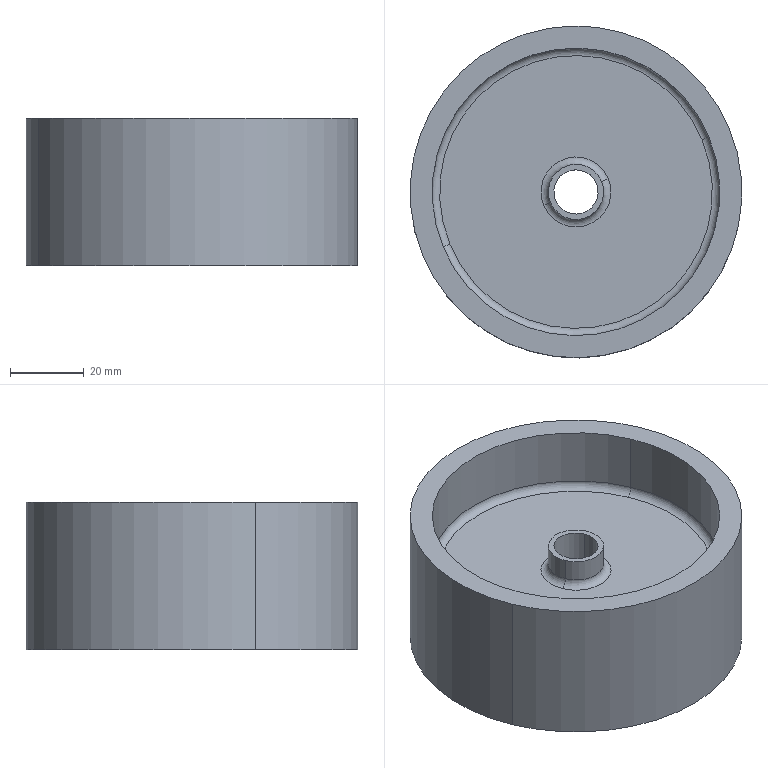Component | SolidWorks | SpringCover-2 | 1 solid | 36 faces | box 90 x 90 x 40 mm | volume 79848 mm3 | cylinder 16 | torus 12 | plane 8 | commonest cylinder face diameters 78 x4 15 x2 86 x2 18 x2 24 x2 12 x2 90 x2
build123d program:
from build123d import *

# Parameters (mm, degrees)
SKETCH1_R           = 45
SKETCH1_R_2         = 39
BOSS_EXTRUDE1_DEPTH = 20
SKETCH2_R           = 40
SKETCH2_R_2         = 6
BOSS_EXTRUDE2_DEPTH = 2
SKETCH3_R           = 12
SKETCH3_R_2         = 9
BOSS_EXTRUDE3_DEPTH = 16
BOSS_EXTRUDE4_START = 8
SKETCH5_R           = 7.5
SKETCH5_R_2         = 6
BOSS_EXTRUDE4_DEPTH = 8
FILLET1_R           = 2


with BuildPart() as part:
    # Sketch1 → Boss-Extrude1 (new, symmetric)
    with BuildSketch(Plane.XY):
        Circle(SKETCH1_R)
        Circle(SKETCH1_R_2, mode=Mode.SUBTRACT)
    extrude(amount=BOSS_EXTRUDE1_DEPTH, both=True)

    # Sketch2 → Boss-Extrude2 (add, symmetric)
    with BuildSketch(Plane.XY):
        Circle(SKETCH2_R)
        Circle(SKETCH2_R_2, mode=Mode.SUBTRACT)
    extrude(amount=BOSS_EXTRUDE2_DEPTH, both=True)

    # Sketch3 → Boss-Extrude3 (add)
    with BuildSketch(Plane.XY.offset(2)):
        Circle(SKETCH3_R)
        Circle(SKETCH3_R_2, mode=Mode.SUBTRACT)
    extrude(amount=BOSS_EXTRUDE3_DEPTH)

    # Sketch4 → Cut-Revolve1 (revolve, cut)
    with BuildSketch(Plane(origin=(0, 0, 0), x_dir=(1, 0, 0), z_dir=(0, 1, 0))):
        Polygon((-43, -14), (-33.035, -14), (-33.287, -20), (-43, -20), align=None)
    revolve(axis=Axis((0, 0, -26.979), (0, 0, 1)), mode=Mode.SUBTRACT)

    # Sketch5 → Boss-Extrude4 (add)
    with BuildSketch(Plane(origin=(0, 0, -2), x_dir=(-1, 0, 0), z_dir=(0, 0, -1)).offset(BOSS_EXTRUDE4_START)):
        with Locations(Location((0, 0, 0), (0, 0, 180))):
            Circle(SKETCH5_R)
        Circle(SKETCH5_R_2, mode=Mode.SUBTRACT)
    extrude(amount=-BOSS_EXTRUDE4_DEPTH)

    # Fillet1
    fillet1_edges = [part.edges().sort_by_distance(p)[0] for p in [
        (-39, 0, 2),
        (-39, 0, -2),
        (-9, 0, 2),
        (-12, 0, 2),
        (-39, 0, 14),
        (-7.5, 0, -2),
    ]]
    fillet(fillet1_edges, radius=FILLET1_R)


solid = part.part

# Placed as in the assembly
solid = solid.moved(Location((-15.928, -1.7, 188), (180, 0, 0)))
STEP:
#1=COLOUR_RGB('',0.7922,0.8196,0.9333);
#2=FILL_AREA_STYLE_COLOUR('',#1);
#3=FILL_AREA_STYLE('',(#2));
#4=SURFACE_STYLE_FILL_AREA(#3);
#5=SURFACE_SIDE_STYLE('',(#4));
#6=SURFACE_STYLE_USAGE(.BOTH.,#5);
#7=PRESENTATION_STYLE_ASSIGNMENT((#6));
#8=CARTESIAN_POINT('',(-1.973,-0.6249,7.323));
#9=VERTEX_POINT('',#8);
#10=CARTESIAN_POINT('',(0.7185,0.491,7.323));
#11=VERTEX_POINT('',#10);
#12=CARTESIAN_POINT('',(-0.6271,-0.06694,7.323));
#13=DIRECTION('',(0.,0.,-1.));
#14=DIRECTION('',(0.9237,0.383,0.));
#15=AXIS2_PLACEMENT_3D('',#12,#13,#14);
#16=CIRCLE('',#15,1.457);
#17=EDGE_CURVE('',#9,#11,#16,.T.);
#18=ORIENTED_EDGE('',*,*,#17,.F.);
#19=CARTESIAN_POINT('',(-2.045,-0.6551,7.244));
#20=VERTEX_POINT('',#19);
#21=CARTESIAN_POINT('',(-1.973,-0.6249,7.244));
#22=DIRECTION('',(0.383,-0.9237,0.));
#23=DIRECTION('',(0.9237,0.383,0.));
#24=AXIS2_PLACEMENT_3D('',#21,#22,#23);
#25=CIRCLE('',#24,0.07874);
#26=EDGE_CURVE('',#9,#20,#25,.T.);
#27=ORIENTED_EDGE('',*,*,#26,.T.);
#28=CARTESIAN_POINT('',(0.7912,0.5212,7.244));
#29=VERTEX_POINT('',#28);
#30=CARTESIAN_POINT('',(-0.6271,-0.06694,7.244));
#31=DIRECTION('',(0.,0.,1.));
#32=DIRECTION('',(0.9237,0.383,0.));
#33=AXIS2_PLACEMENT_3D('',#30,#31,#32);
#34=CIRCLE('',#33,1.535);
#35=EDGE_CURVE('',#29,#20,#34,.T.);
#36=ORIENTED_EDGE('',*,*,#35,.F.);
#37=CARTESIAN_POINT('',(0.7185,0.491,7.244));
#38=DIRECTION('',(-0.383,0.9237,0.));
#39=DIRECTION('',(-0.9237,-0.383,0.));
#40=AXIS2_PLACEMENT_3D('',#37,#38,#39);
#41=CIRCLE('',#40,0.07874);
#42=EDGE_CURVE('',#11,#29,#41,.T.);
#43=ORIENTED_EDGE('',*,*,#42,.F.);
#44=EDGE_LOOP('',(#18,#27,#36,#43));
#45=FACE_OUTER_BOUND('',#44,.T.);
#46=CARTESIAN_POINT('',(-0.6271,-0.06694,7.244));
#47=DIRECTION('',(0.,0.,-1.));
#48=DIRECTION('',(0.9237,0.383,0.));
#49=AXIS2_PLACEMENT_3D('',#46,#47,#48);
#50=TOROIDAL_SURFACE('',#49,1.457,0.07874);
#51=ADVANCED_FACE('',(#45),#50,.F.);
#52=CARTESIAN_POINT('',(0.7912,0.5212,6.929));
#53=VERTEX_POINT('',#52);
#54=CARTESIAN_POINT('',(-2.045,-0.6551,6.929));
#55=VERTEX_POINT('',#54);
#56=CARTESIAN_POINT('',(-0.6271,-0.06694,6.929));
#57=DIRECTION('',(0.,0.,-1.));
#58=DIRECTION('',(-0.9237,-0.383,0.));
#59=AXIS2_PLACEMENT_3D('',#56,#57,#58);
#60=CIRCLE('',#59,1.535);
#61=EDGE_CURVE('',#53,#55,#60,.T.);
#62=ORIENTED_EDGE('',*,*,#61,.F.);
#63=CARTESIAN_POINT('',(0.864,0.5514,6.85));
#64=VERTEX_POINT('',#63);
#65=CARTESIAN_POINT('',(0.864,0.5514,6.929));
#66=DIRECTION('',(0.383,-0.9237,0.));
#67=DIRECTION('',(0.9237,0.383,0.));
#68=AXIS2_PLACEMENT_3D('',#65,#66,#67);
#69=CIRCLE('',#68,0.07874);
#70=EDGE_CURVE('',#53,#64,#69,.T.);
#71=ORIENTED_EDGE('',*,*,#70,.T.);
#72=CARTESIAN_POINT('',(-2.118,-0.6852,6.85));
#73=VERTEX_POINT('',#72);
#74=CARTESIAN_POINT('',(-0.6271,-0.06694,6.85));
#75=DIRECTION('',(0.,0.,1.));
#76=DIRECTION('',(-0.9237,-0.383,0.));
#77=AXIS2_PLACEMENT_3D('',#74,#75,#76);
#78=CIRCLE('',#77,1.614);
#79=EDGE_CURVE('',#73,#64,#78,.T.);
#80=ORIENTED_EDGE('',*,*,#79,.F.);
#81=CARTESIAN_POINT('',(-2.118,-0.6852,6.929));
#82=DIRECTION('',(-0.383,0.9237,0.));
#83=DIRECTION('',(-0.9237,-0.383,0.));
#84=AXIS2_PLACEMENT_3D('',#81,#82,#83);
#85=CIRCLE('',#84,0.07874);
#86=EDGE_CURVE('',#55,#73,#85,.T.);
#87=ORIENTED_EDGE('',*,*,#86,.F.);
#88=EDGE_LOOP('',(#62,#71,#80,#87));
#89=FACE_OUTER_BOUND('',#88,.T.);
#90=CARTESIAN_POINT('',(-0.6271,-0.06694,6.929));
#91=DIRECTION('',(0.,0.,1.));
#92=DIRECTION('',(-0.9237,-0.383,0.));
#93=AXIS2_PLACEMENT_3D('',#90,#91,#92);
#94=TOROIDAL_SURFACE('',#93,1.614,0.07874);
#95=ADVANCED_FACE('',(#89),#94,.T.);
#96=CARTESIAN_POINT('',(-0.8817,-0.1725,7.323));
#97=VERTEX_POINT('',#96);
#98=CARTESIAN_POINT('',(-0.3725,0.03863,7.323));
#99=VERTEX_POINT('',#98);
#100=CARTESIAN_POINT('',(-0.6271,-0.06694,7.323));
#101=DIRECTION('',(0.,0.,-1.));
#102=DIRECTION('',(0.9237,0.383,0.));
#103=AXIS2_PLACEMENT_3D('',#100,#101,#102);
#104=CIRCLE('',#103,0.2756);
#105=EDGE_CURVE('',#97,#99,#104,.T.);
#106=ORIENTED_EDGE('',*,*,#105,.F.);
#107=CARTESIAN_POINT('',(-0.9544,-0.2027,7.244));
#108=VERTEX_POINT('',#107);
#109=CARTESIAN_POINT('',(-0.8817,-0.1725,7.244));
#110=DIRECTION('',(0.383,-0.9237,0.));
#111=DIRECTION('',(0.9237,0.383,0.));
#112=AXIS2_PLACEMENT_3D('',#109,#110,#111);
#113=CIRCLE('',#112,0.07874);
#114=EDGE_CURVE('',#97,#108,#113,.T.);
#115=ORIENTED_EDGE('',*,*,#114,.T.);
#116=CARTESIAN_POINT('',(-0.2998,0.06879,7.244));
#117=VERTEX_POINT('',#116);
#118=CARTESIAN_POINT('',(-0.6271,-0.06694,7.244));
#119=DIRECTION('',(0.,0.,1.));
#120=DIRECTION('',(0.9237,0.383,0.));
#121=AXIS2_PLACEMENT_3D('',#118,#119,#120);
#122=CIRCLE('',#121,0.3543);
#123=EDGE_CURVE('',#117,#108,#122,.T.);
#124=ORIENTED_EDGE('',*,*,#123,.F.);
#125=CARTESIAN_POINT('',(-0.3725,0.03863,7.244));
#126=DIRECTION('',(-0.383,0.9237,0.));
#127=DIRECTION('',(-0.9237,-0.383,0.));
#128=AXIS2_PLACEMENT_3D('',#125,#126,#127);
#129=CIRCLE('',#128,0.07874);
#130=EDGE_CURVE('',#99,#117,#129,.T.);
#131=ORIENTED_EDGE('',*,*,#130,.F.);
#132=EDGE_LOOP('',(#106,#115,#124,#131));
#133=FACE_OUTER_BOUND('',#132,.T.);
#134=CARTESIAN_POINT('',(-0.6271,-0.06694,7.244));
#135=DIRECTION('',(0.,0.,-1.));
#136=DIRECTION('',(0.9237,0.383,0.));
#137=AXIS2_PLACEMENT_3D('',#134,#135,#136);
#138=TOROIDAL_SURFACE('',#137,0.2756,0.07874);
#139=ADVANCED_FACE('',(#133),#138,.F.);
#140=CARTESIAN_POINT('',(-1.063,-0.2479,7.244));
#141=VERTEX_POINT('',#140);
#142=CARTESIAN_POINT('',(-0.1907,0.114,7.244));
#143=VERTEX_POINT('',#142);
#144=CARTESIAN_POINT('',(-0.6271,-0.06694,7.244));
#145=DIRECTION('',(0.,0.,-1.));
#146=DIRECTION('',(0.9237,0.383,0.));
#147=AXIS2_PLACEMENT_3D('',#144,#145,#146);
#148=CIRCLE('',#147,0.4724);
#149=EDGE_CURVE('',#141,#143,#148,.T.);
#150=ORIENTED_EDGE('',*,*,#149,.F.);
#151=CARTESIAN_POINT('',(-1.136,-0.2781,7.323));
#152=VERTEX_POINT('',#151);
#153=CARTESIAN_POINT('',(-1.136,-0.2781,7.244));
#154=DIRECTION('',(0.383,-0.9237,0.));
#155=DIRECTION('',(0.9237,0.383,0.));
#156=AXIS2_PLACEMENT_3D('',#153,#154,#155);
#157=CIRCLE('',#156,0.07874);
#158=EDGE_CURVE('',#141,#152,#157,.T.);
#159=ORIENTED_EDGE('',*,*,#158,.T.);
#160=CARTESIAN_POINT('',(-0.1179,0.1442,7.323));
#161=VERTEX_POINT('',#160);
#162=CARTESIAN_POINT('',(-0.6271,-0.06694,7.323));
#163=DIRECTION('',(0.,0.,1.));
#164=DIRECTION('',(0.9237,0.383,0.));
#165=AXIS2_PLACEMENT_3D('',#162,#163,#164);
#166=CIRCLE('',#165,0.5512);
#167=EDGE_CURVE('',#161,#152,#166,.T.);
#168=ORIENTED_EDGE('',*,*,#167,.F.);
#169=CARTESIAN_POINT('',(-0.1179,0.1442,7.244));
#170=DIRECTION('',(-0.383,0.9237,0.));
#171=DIRECTION('',(-0.9237,-0.383,0.));
#172=AXIS2_PLACEMENT_3D('',#169,#170,#171);
#173=CIRCLE('',#172,0.07874);
#174=EDGE_CURVE('',#143,#161,#173,.T.);
#175=ORIENTED_EDGE('',*,*,#174,.F.);
#176=EDGE_LOOP('',(#150,#159,#168,#175));
#177=FACE_OUTER_BOUND('',#176,.T.);
#178=CARTESIAN_POINT('',(-0.6271,-0.06694,7.244));
#179=DIRECTION('',(0.,0.,-1.));
#180=DIRECTION('',(0.9237,0.383,0.));
#181=AXIS2_PLACEMENT_3D('',#178,#179,#180);
#182=TOROIDAL_SURFACE('',#181,0.5512,0.07874);
#183=ADVANCED_FACE('',(#177),#182,.F.);
#184=CARTESIAN_POINT('',(-2.045,-0.6551,7.559));
#185=VERTEX_POINT('',#184);
#186=CARTESIAN_POINT('',(0.7912,0.5212,7.559));
#187=VERTEX_POINT('',#186);
#188=CARTESIAN_POINT('',(-0.6271,-0.06694,7.559));
#189=DIRECTION('',(0.,0.,-1.));
#190=DIRECTION('',(0.9237,0.383,0.));
#191=AXIS2_PLACEMENT_3D('',#188,#189,#190);
#192=CIRCLE('',#191,1.535);
#193=EDGE_CURVE('',#185,#187,#192,.T.);
#194=ORIENTED_EDGE('',*,*,#193,.F.);
#195=CARTESIAN_POINT('',(-1.973,-0.6249,7.48));
#196=VERTEX_POINT('',#195);
#197=CARTESIAN_POINT('',(-1.973,-0.6249,7.559));
#198=DIRECTION('',(0.383,-0.9237,0.));
#199=DIRECTION('',(0.9237,0.383,0.));
#200=AXIS2_PLACEMENT_3D('',#197,#198,#199);
#201=CIRCLE('',#200,0.07874);
#202=EDGE_CURVE('',#185,#196,#201,.T.);
#203=ORIENTED_EDGE('',*,*,#202,.T.);
#204=CARTESIAN_POINT('',(0.7185,0.491,7.48));
#205=VERTEX_POINT('',#204);
#206=CARTESIAN_POINT('',(-0.6271,-0.06694,7.48));
#207=DIRECTION('',(0.,0.,1.));
#208=DIRECTION('',(0.9237,0.383,0.));
#209=AXIS2_PLACEMENT_3D('',#206,#207,#208);
#210=CIRCLE('',#209,1.457);
#211=EDGE_CURVE('',#205,#196,#210,.T.);
#212=ORIENTED_EDGE('',*,*,#211,.F.);
#213=CARTESIAN_POINT('',(0.7185,0.491,7.559));
#214=DIRECTION('',(-0.383,0.9237,0.));
#215=DIRECTION('',(-0.9237,-0.383,0.));
#216=AXIS2_PLACEMENT_3D('',#213,#214,#215);
#217=CIRCLE('',#216,0.07874);
#218=EDGE_CURVE('',#187,#205,#217,.T.);
#219=ORIENTED_EDGE('',*,*,#218,.F.);
#220=EDGE_LOOP('',(#194,#203,#212,#219));
#221=FACE_OUTER_BOUND('',#220,.T.);
#222=CARTESIAN_POINT('',(-0.6271,-0.06694,7.559));
#223=DIRECTION('',(0.,0.,-1.));
#224=DIRECTION('',(0.9237,0.383,0.));
#225=AXIS2_PLACEMENT_3D('',#222,#223,#224);
#226=TOROIDAL_SURFACE('',#225,1.457,0.07874);
#227=ADVANCED_FACE('',(#221),#226,.F.);
#228=CARTESIAN_POINT('',(-0.9726,-0.2102,7.48));
#229=VERTEX_POINT('',#228);
#230=CARTESIAN_POINT('',(-0.2816,0.07633,7.48));
#231=VERTEX_POINT('',#230);
#232=CARTESIAN_POINT('',(-0.6271,-0.06694,7.48));
#233=DIRECTION('',(0.,0.,-1.));
#234=DIRECTION('',(0.9237,0.383,0.));
#235=AXIS2_PLACEMENT_3D('',#232,#233,#234);
#236=CIRCLE('',#235,0.374);
#237=EDGE_CURVE('',#229,#231,#236,.T.);
#238=ORIENTED_EDGE('',*,*,#237,.F.);
#239=CARTESIAN_POINT('',(-0.8998,-0.18,7.559));
#240=VERTEX_POINT('',#239);
#241=CARTESIAN_POINT('',(-0.9726,-0.2102,7.559));
#242=DIRECTION('',(0.383,-0.9237,0.));
#243=DIRECTION('',(0.9237,0.383,0.));
#244=AXIS2_PLACEMENT_3D('',#241,#242,#243);
#245=CIRCLE('',#244,0.07874);
#246=EDGE_CURVE('',#229,#240,#245,.T.);
#247=ORIENTED_EDGE('',*,*,#246,.T.);
#248=CARTESIAN_POINT('',(-0.3543,0.04617,7.559));
#249=VERTEX_POINT('',#248);
#250=CARTESIAN_POINT('',(-0.6271,-0.06694,7.559));
#251=DIRECTION('',(0.,0.,1.));
#252=DIRECTION('',(0.9237,0.383,0.));
#253=AXIS2_PLACEMENT_3D('',#250,#251,#252);
#254=CIRCLE('',#253,0.2953);
#255=EDGE_CURVE('',#249,#240,#254,.T.);
#256=ORIENTED_EDGE('',*,*,#255,.F.);
#257=CARTESIAN_POINT('',(-0.2816,0.07633,7.559));
#258=DIRECTION('',(-0.383,0.9237,0.));
#259=DIRECTION('',(-0.9237,-0.383,0.));
#260=AXIS2_PLACEMENT_3D('',#257,#258,#259);
#261=CIRCLE('',#260,0.07874);
#262=EDGE_CURVE('',#231,#249,#261,.T.);
#263=ORIENTED_EDGE('',*,*,#262,.F.);
#264=EDGE_LOOP('',(#238,#247,#256,#263));
#265=FACE_OUTER_BOUND('',#264,.T.);
#266=CARTESIAN_POINT('',(-0.6271,-0.06694,7.559));
#267=DIRECTION('',(0.,0.,-1.));
#268=DIRECTION('',(0.9237,0.383,0.));
#269=AXIS2_PLACEMENT_3D('',#266,#267,#268);
#270=TOROIDAL_SURFACE('',#269,0.374,0.07874);
#271=ADVANCED_FACE('',(#265),#270,.F.);
#272=CARTESIAN_POINT('',(-0.8998,-0.18,7.795));
#273=VERTEX_POINT('',#272);
#274=CARTESIAN_POINT('',(-0.3543,0.04617,7.795));
#275=VERTEX_POINT('',#274);
#276=CARTESIAN_POINT('',(-0.6271,-0.06694,7.795));
#277=DIRECTION('',(0.,0.,1.));
#278=DIRECTION('',(-0.9237,-0.383,0.));
#279=AXIS2_PLACEMENT_3D('',#276,#277,#278);
#280=CIRCLE('',#279,0.2953);
#281=EDGE_CURVE('',#273,#275,#280,.T.);
#282=ORIENTED_EDGE('',*,*,#281,.F.);
#283=CARTESIAN_POINT('',(-0.8998,-0.18,7.795));
#284=DIRECTION('',(0.,0.,-1.));
#285=VECTOR('',#284,39.37);
#286=LINE('',#283,#285);
#287=EDGE_CURVE('',#273,#240,#286,.T.);
#288=ORIENTED_EDGE('',*,*,#287,.T.);
#289=CARTESIAN_POINT('',(-0.6271,-0.06694,7.559));
#290=DIRECTION('',(0.,0.,1.));
#291=DIRECTION('',(0.9237,0.383,0.));
#292=AXIS2_PLACEMENT_3D('',#289,#290,#291);
#293=CIRCLE('',#292,0.2953);
#294=EDGE_CURVE('',#240,#249,#293,.T.);
#295=ORIENTED_EDGE('',*,*,#294,.T.);
#296=CARTESIAN_POINT('',(-0.3543,0.04617,7.795));
#297=DIRECTION('',(0.,0.,-1.));
#298=VECTOR('',#297,39.37);
#299=LINE('',#296,#298);
#300=EDGE_CURVE('',#275,#249,#299,.T.);
#301=ORIENTED_EDGE('',*,*,#300,.F.);
#302=EDGE_LOOP('',(#282,#288,#295,#301));
#303=FACE_OUTER_BOUND('',#302,.T.);
#304=CARTESIAN_POINT('',(-0.6271,-0.06694,7.795));
#305=DIRECTION('',(0.,0.,-1.));
#306=DIRECTION('',(0.9237,0.383,0.));
#307=AXIS2_PLACEMENT_3D('',#304,#305,#306);
#308=CYLINDRICAL_SURFACE('',#307,0.2953);
#309=ADVANCED_FACE('',(#303),#308,.T.);
#310=CARTESIAN_POINT('',(0.9367,0.5815,6.614));
#311=VERTEX_POINT('',#310);
#312=CARTESIAN_POINT('',(-2.191,-0.7154,6.614));
#313=VERTEX_POINT('',#312);
#314=CARTESIAN_POINT('',(-0.6271,-0.06694,6.614));
#315=DIRECTION('',(0.,0.,1.));
#316=DIRECTION('',(-0.9237,-0.383,0.));
#317=AXIS2_PLACEMENT_3D('',#314,#315,#316);
#318=CIRCLE('',#317,1.693);
#319=EDGE_CURVE('',#311,#313,#318,.T.);
#320=ORIENTED_EDGE('',*,*,#319,.F.);
#321=CARTESIAN_POINT('',(0.9367,0.5815,6.85));
#322=VERTEX_POINT('',#321);
#323=CARTESIAN_POINT('',(0.9367,0.5815,8.464));
#324=DIRECTION('',(0.,0.,1.));
#325=VECTOR('',#324,39.37);
#326=LINE('',#323,#325);
#327=EDGE_CURVE('',#311,#322,#326,.T.);
#328=ORIENTED_EDGE('',*,*,#327,.T.);
#329=CARTESIAN_POINT('',(-2.191,-0.7154,6.85));
#330=VERTEX_POINT('',#329);
#331=CARTESIAN_POINT('',(-0.6271,-0.06694,6.85));
#332=DIRECTION('',(0.,0.,1.));
#333=DIRECTION('',(-0.9237,-0.383,0.));
#334=AXIS2_PLACEMENT_3D('',#331,#332,#333);
#335=CIRCLE('',#334,1.693);
#336=EDGE_CURVE('',#322,#330,#335,.T.);
#337=ORIENTED_EDGE('',*,*,#336,.T.);
#338=CARTESIAN_POINT('',(-2.191,-0.7154,8.464));
#339=DIRECTION('',(0.,0.,1.));
#340=VECTOR('',#339,39.37);
#341=LINE('',#338,#340);
#342=EDGE_CURVE('',#313,#330,#341,.T.);
#343=ORIENTED_EDGE('',*,*,#342,.F.);
#344=EDGE_LOOP('',(#320,#328,#337,#343));
#345=FACE_OUTER_BOUND('',#344,.T.);
#346=CARTESIAN_POINT('',(-0.6271,-0.06694,8.464));
#347=DIRECTION('',(0.,0.,1.));
#348=DIRECTION('',(-0.9237,-0.383,0.));
#349=AXIS2_PLACEMENT_3D('',#346,#347,#348);
#350=CYLINDRICAL_SURFACE('',#349,1.693);
#351=ADVANCED_FACE('',(#345),#350,.F.);
#352=CARTESIAN_POINT('',(-0.9544,-0.2027,6.693));
#353=VERTEX_POINT('',#352);
#354=CARTESIAN_POINT('',(-0.2998,0.06879,6.693));
#355=VERTEX_POINT('',#354);
#356=CARTESIAN_POINT('',(-0.6271,-0.06694,6.693));
#357=DIRECTION('',(0.,0.,-1.));
#358=DIRECTION('',(0.9237,0.383,0.));
#359=AXIS2_PLACEMENT_3D('',#356,#357,#358);
#360=CIRCLE('',#359,0.3543);
#361=EDGE_CURVE('',#353,#355,#360,.T.);
#362=ORIENTED_EDGE('',*,*,#361,.T.);
#363=CARTESIAN_POINT('',(-0.2998,0.06879,6.693));
#364=DIRECTION('',(0.,0.,1.));
#365=VECTOR('',#364,39.37);
#366=LINE('',#363,#365);
#367=EDGE_CURVE('',#355,#117,#366,.T.);
#368=ORIENTED_EDGE('',*,*,#367,.T.);
#369=ORIENTED_EDGE('',*,*,#123,.T.);
#370=CARTESIAN_POINT('',(-0.9544,-0.2027,6.693));
#371=DIRECTION('',(0.,0.,1.));
#372=VECTOR('',#371,39.37);
#373=LINE('',#370,#372);
#374=EDGE_CURVE('',#353,#108,#373,.T.);
#375=ORIENTED_EDGE('',*,*,#374,.F.);
#376=EDGE_LOOP('',(#362,#368,#369,#375));
#377=FACE_OUTER_BOUND('',#376,.T.);
#378=CARTESIAN_POINT('',(-0.6271,-0.06694,6.693));
#379=DIRECTION('',(0.,0.,1.));
#380=DIRECTION('',(-0.9237,-0.383,0.));
#381=AXIS2_PLACEMENT_3D('',#378,#379,#380);
#382=CYLINDRICAL_SURFACE('',#381,0.3543);
#383=ADVANCED_FACE('',(#377),#382,.F.);
#384=CARTESIAN_POINT('',(-0.1907,0.114,6.693));
#385=VERTEX_POINT('',#384);
#386=CARTESIAN_POINT('',(-1.063,-0.2479,6.693));
#387=VERTEX_POINT('',#386);
#388=CARTESIAN_POINT('',(-0.6271,-0.06694,6.693));
#389=DIRECTION('',(0.,0.,-1.));
#390=DIRECTION('',(0.9237,0.383,0.));
#391=AXIS2_PLACEMENT_3D('',#388,#389,#390);
#392=CIRCLE('',#391,0.4724);
#393=EDGE_CURVE('',#385,#387,#392,.T.);
#394=ORIENTED_EDGE('',*,*,#393,.F.);
#395=CARTESIAN_POINT('',(-0.1907,0.114,6.693));
#396=DIRECTION('',(0.,0.,1.));
#397=VECTOR('',#396,39.37);
#398=LINE('',#395,#397);
#399=EDGE_CURVE('',#385,#143,#398,.T.);
#400=ORIENTED_EDGE('',*,*,#399,.T.);
#401=CARTESIAN_POINT('',(-0.6271,-0.06694,7.244));
#402=DIRECTION('',(0.,0.,-1.));
#403=DIRECTION('',(0.9237,0.383,0.));
#404=AXIS2_PLACEMENT_3D('',#401,#402,#403);
#405=CIRCLE('',#404,0.4724);
#406=EDGE_CURVE('',#143,#141,#405,.T.);
#407=ORIENTED_EDGE('',*,*,#406,.T.);
#408=CARTESIAN_POINT('',(-1.063,-0.2479,6.693));
#409=DIRECTION('',(0.,0.,1.));
#410=VECTOR('',#409,39.37);
#411=LINE('',#408,#410);
#412=EDGE_CURVE('',#387,#141,#411,.T.);
#413=ORIENTED_EDGE('',*,*,#412,.F.);
#414=EDGE_LOOP('',(#394,#400,#407,#413));
#415=FACE_OUTER_BOUND('',#414,.T.);
#416=CARTESIAN_POINT('',(-0.6271,-0.06694,6.693));
#417=DIRECTION('',(0.,0.,1.));
#418=DIRECTION('',(-0.9237,-0.383,0.));
#419=AXIS2_PLACEMENT_3D('',#416,#417,#418);
#420=CYLINDRICAL_SURFACE('',#419,0.4724);
#421=ADVANCED_FACE('',(#415),#420,.T.);
#422=CARTESIAN_POINT('',(-0.8453,-0.1574,7.323));
#423=VERTEX_POINT('',#422);
#424=CARTESIAN_POINT('',(-0.4089,0.02355,7.323));
#425=VERTEX_POINT('',#424);
#426=CARTESIAN_POINT('',(-0.6271,-0.06694,7.323));
#427=DIRECTION('',(0.,0.,-1.));
#428=DIRECTION('',(0.9237,0.383,0.));
#429=AXIS2_PLACEMENT_3D('',#426,#427,#428);
#430=CIRCLE('',#429,0.2362);
#431=EDGE_CURVE('',#423,#425,#430,.T.);
#432=ORIENTED_EDGE('',*,*,#431,.T.);
#433=CARTESIAN_POINT('',(-0.4089,0.02355,7.795));
#434=VERTEX_POINT('',#433);
#435=CARTESIAN_POINT('',(-0.4089,0.02355,7.323));
#436=DIRECTION('',(0.,0.,1.));
#437=VECTOR('',#436,39.37);
#438=LINE('',#435,#437);
#439=EDGE_CURVE('',#425,#434,#438,.T.);
#440=ORIENTED_EDGE('',*,*,#439,.T.);
#441=CARTESIAN_POINT('',(-0.8453,-0.1574,7.795));
#442=VERTEX_POINT('',#441);
#443=CARTESIAN_POINT('',(-0.6271,-0.06694,7.795));
#444=DIRECTION('',(0.,0.,1.));
#445=DIRECTION('',(-0.9237,-0.383,0.));
#446=AXIS2_PLACEMENT_3D('',#443,#444,#445);
#447=CIRCLE('',#446,0.2362);
#448=EDGE_CURVE('',#434,#442,#447,.T.);
#449=ORIENTED_EDGE('',*,*,#448,.T.);
#450=CARTESIAN_POINT('',(-0.8453,-0.1574,7.323));
#451=DIRECTION('',(0.,0.,1.));
#452=VECTOR('',#451,39.37);
#453=LINE('',#450,#452);
#454=EDGE_CURVE('',#423,#442,#453,.T.);
#455=ORIENTED_EDGE('',*,*,#454,.F.);
#456=EDGE_LOOP('',(#432,#440,#449,#455));
#457=FACE_OUTER_BOUND('',#456,.T.);
#458=CARTESIAN_POINT('',(-0.6271,-0.06694,7.323));
#459=DIRECTION('',(0.,0.,1.));
#460=DIRECTION('',(-0.9237,-0.383,0.));
#461=AXIS2_PLACEMENT_3D('',#458,#459,#460);
#462=CYLINDRICAL_SURFACE('',#461,0.2362);
#463=ADVANCED_FACE('',(#457),#462,.F.);
#464=CARTESIAN_POINT('',(-0.6271,-0.06694,6.929));
#465=DIRECTION('',(0.,0.,-1.));
#466=DIRECTION('',(-0.9237,-0.383,0.));
#467=AXIS2_PLACEMENT_3D('',#464,#465,#466);
#468=CIRCLE('',#467,1.535);
#469=EDGE_CURVE('',#55,#53,#468,.T.);
#470=ORIENTED_EDGE('',*,*,#469,.T.);
#471=CARTESIAN_POINT('',(0.7912,0.5212,6.614));
#472=DIRECTION('',(0.,0.,1.));
#473=VECTOR('',#472,39.37);
#474=LINE('',#471,#473);
#475=EDGE_CURVE('',#53,#29,#474,.T.);
#476=ORIENTED_EDGE('',*,*,#475,.T.);
#477=ORIENTED_EDGE('',*,*,#35,.T.);
#478=CARTESIAN_POINT('',(-2.045,-0.6551,6.614));
#479=DIRECTION('',(0.,0.,1.));
#480=VECTOR('',#479,39.37);
#481=LINE('',#478,#480);
#482=EDGE_CURVE('',#55,#20,#481,.T.);
#483=ORIENTED_EDGE('',*,*,#482,.F.);
#484=EDGE_LOOP('',(#470,#476,#477,#483));
#485=FACE_OUTER_BOUND('',#484,.T.);
#486=CARTESIAN_POINT('',(-0.6271,-0.06694,6.614));
#487=DIRECTION('',(0.,0.,1.));
#488=DIRECTION('',(-0.9237,-0.383,0.));
#489=AXIS2_PLACEMENT_3D('',#486,#487,#488);
#490=CYLINDRICAL_SURFACE('',#489,1.535);
#491=ADVANCED_FACE('',(#485),#490,.F.);
#492=CARTESIAN_POINT('',(1.009,0.6117,6.614));
#493=VERTEX_POINT('',#492);
#494=CARTESIAN_POINT('',(-2.264,-0.7456,6.614));
#495=VERTEX_POINT('',#494);
#496=CARTESIAN_POINT('',(-0.6271,-0.06694,6.614));
#497=DIRECTION('',(0.,0.,-1.));
#498=DIRECTION('',(0.9237,0.383,0.));
#499=AXIS2_PLACEMENT_3D('',#496,#497,#498);
#500=CIRCLE('',#499,1.772);
#501=EDGE_CURVE('',#493,#495,#500,.T.);
#502=ORIENTED_EDGE('',*,*,#501,.F.);
#503=CARTESIAN_POINT('',(1.009,0.6117,8.189));
#504=VERTEX_POINT('',#503);
#505=CARTESIAN_POINT('',(1.009,0.6117,6.614));
#506=DIRECTION('',(0.,0.,1.));
#507=VECTOR('',#506,39.37);
#508=LINE('',#505,#507);
#509=EDGE_CURVE('',#493,#504,#508,.T.);
#510=ORIENTED_EDGE('',*,*,#509,.T.);
#511=CARTESIAN_POINT('',(-2.264,-0.7456,8.189));
#512=VERTEX_POINT('',#511);
#513=CARTESIAN_POINT('',(-0.6271,-0.06694,8.189));
#514=DIRECTION('',(0.,0.,-1.));
#515=DIRECTION('',(0.9237,0.383,0.));
#516=AXIS2_PLACEMENT_3D('',#513,#514,#515);
#517=CIRCLE('',#516,1.772);
#518=EDGE_CURVE('',#504,#512,#517,.T.);
#519=ORIENTED_EDGE('',*,*,#518,.T.);
#520=CARTESIAN_POINT('',(-2.264,-0.7456,6.614));
#521=DIRECTION('',(0.,0.,1.));
#522=VECTOR('',#521,39.37);
#523=LINE('',#520,#522);
#524=EDGE_CURVE('',#495,#512,#523,.T.);
#525=ORIENTED_EDGE('',*,*,#524,.F.);
#526=EDGE_LOOP('',(#502,#510,#519,#525));
#527=FACE_OUTER_BOUND('',#526,.T.);
#528=CARTESIAN_POINT('',(-0.6271,-0.06694,6.614));
#529=DIRECTION('',(0.,0.,1.));
#530=DIRECTION('',(-0.9237,-0.383,0.));
#531=AXIS2_PLACEMENT_3D('',#528,#529,#530);
#532=CYLINDRICAL_SURFACE('',#531,1.772);
#533=ADVANCED_FACE('',(#527),#532,.T.);
#534=ORIENTED_EDGE('',*,*,#193,.T.);
#535=CARTESIAN_POINT('',(0.7912,0.5212,8.189));
#536=VERTEX_POINT('',#535);
#537=CARTESIAN_POINT('',(0.7912,0.5212,6.614));
#538=DIRECTION('',(0.,0.,1.));
#539=VECTOR('',#538,39.37);
#540=LINE('',#537,#539);
#541=EDGE_CURVE('',#187,#536,#540,.T.);
#542=ORIENTED_EDGE('',*,*,#541,.T.);
#543=CARTESIAN_POINT('',(-2.045,-0.6551,8.189));
#544=VERTEX_POINT('',#543);
#545=CARTESIAN_POINT('',(-0.6271,-0.06694,8.189));
#546=DIRECTION('',(0.,0.,-1.));
#547=DIRECTION('',(0.9237,0.383,0.));
#548=AXIS2_PLACEMENT_3D('',#545,#546,#547);
#549=CIRCLE('',#548,1.535);
#550=EDGE_CURVE('',#544,#536,#549,.T.);
#551=ORIENTED_EDGE('',*,*,#550,.F.);
#552=CARTESIAN_POINT('',(-2.045,-0.6551,6.614));
#553=DIRECTION('',(0.,0.,1.));
#554=VECTOR('',#553,39.37);
#555=LINE('',#552,#554);
#556=EDGE_CURVE('',#185,#544,#555,.T.);
#557=ORIENTED_EDGE('',*,*,#556,.F.);
#558=EDGE_LOOP('',(#534,#542,#551,#557));
#559=FACE_OUTER_BOUND('',#558,.T.);
#560=CARTESIAN_POINT('',(-0.6271,-0.06694,6.614));
#561=DIRECTION('',(0.,0.,1.));
#562=DIRECTION('',(-0.9237,-0.383,0.));
#563=AXIS2_PLACEMENT_3D('',#560,#561,#562);
#564=CYLINDRICAL_SURFACE('',#563,1.535);
#565=ADVANCED_FACE('',(#559),#564,.F.);
#566=CARTESIAN_POINT('',(-0.6271,-0.06694,7.48));
#567=DIRECTION('',(0.,0.,-1.));
#568=DIRECTION('',(0.9237,0.383,0.));
#569=AXIS2_PLACEMENT_3D('',#566,#567,#568);
#570=CIRCLE('',#569,0.374);
#571=EDGE_CURVE('',#231,#229,#570,.T.);
#572=ORIENTED_EDGE('',*,*,#571,.T.);
#573=ORIENTED_EDGE('',*,*,#237,.T.);
#574=EDGE_LOOP('',(#572,#573));
#575=FACE_BOUND('',#574,.T.);
#576=ORIENTED_EDGE('',*,*,#211,.T.);
#577=CARTESIAN_POINT('',(-0.6271,-0.06694,7.48));
#578=DIRECTION('',(0.,0.,1.));
#579=DIRECTION('',(0.9237,0.383,0.));
#580=AXIS2_PLACEMENT_3D('',#577,#578,#579);
#581=CIRCLE('',#580,1.457);
#582=EDGE_CURVE('',#196,#205,#581,.T.);
#583=ORIENTED_EDGE('',*,*,#582,.T.);
#584=EDGE_LOOP('',(#576,#583));
#585=FACE_OUTER_BOUND('',#584,.T.);
#586=CARTESIAN_POINT('',(-0.6271,-0.06694,7.48));
#587=DIRECTION('',(0.,0.,-1.));
#588=DIRECTION('',(0.9237,0.383,0.));
#589=AXIS2_PLACEMENT_3D('',#586,#587,#588);
#590=PLANE('',#589);
#591=ADVANCED_FACE('',(#575,#585),#590,.F.);
#592=ORIENTED_EDGE('',*,*,#167,.T.);
#593=CARTESIAN_POINT('',(-0.6271,-0.06694,7.323));
#594=DIRECTION('',(0.,0.,1.));
#595=DIRECTION('',(0.9237,0.383,0.));
#596=AXIS2_PLACEMENT_3D('',#593,#594,#595);
#597=CIRCLE('',#596,0.5512);
#598=EDGE_CURVE('',#152,#161,#597,.T.);
#599=ORIENTED_EDGE('',*,*,#598,.T.);
#600=EDGE_LOOP('',(#592,#599));
#601=FACE_BOUND('',#600,.T.);
#602=CARTESIAN_POINT('',(-0.6271,-0.06694,7.323));
#603=DIRECTION('',(0.,0.,-1.));
#604=DIRECTION('',(0.9237,0.383,0.));
#605=AXIS2_PLACEMENT_3D('',#602,#603,#604);
#606=CIRCLE('',#605,1.457);
#607=EDGE_CURVE('',#11,#9,#606,.T.);
#608=ORIENTED_EDGE('',*,*,#607,.T.);
#609=ORIENTED_EDGE('',*,*,#17,.T.);
#610=EDGE_LOOP('',(#608,#609));
#611=FACE_OUTER_BOUND('',#610,.T.);
#612=CARTESIAN_POINT('',(-0.6271,-0.06694,7.323));
#613=DIRECTION('',(0.,0.,-1.));
#614=DIRECTION('',(0.9237,0.383,0.));
#615=AXIS2_PLACEMENT_3D('',#612,#613,#614);
#616=PLANE('',#615);
#617=ADVANCED_FACE('',(#601,#611),#616,.T.);
#618=ORIENTED_EDGE('',*,*,#541,.F.);
#619=CARTESIAN_POINT('',(-0.6271,-0.06694,7.559));
#620=DIRECTION('',(0.,0.,-1.));
#621=DIRECTION('',(0.9237,0.383,0.));
#622=AXIS2_PLACEMENT_3D('',#619,#620,#621);
#623=CIRCLE('',#622,1.535);
#624=EDGE_CURVE('',#187,#185,#623,.T.);
#625=ORIENTED_EDGE('',*,*,#624,.T.);
#626=ORIENTED_EDGE('',*,*,#556,.T.);
#627=CARTESIAN_POINT('',(-0.6271,-0.06694,8.189));
#628=DIRECTION('',(0.,0.,-1.));
#629=DIRECTION('',(0.9237,0.383,0.));
#630=AXIS2_PLACEMENT_3D('',#627,#628,#629);
#631=CIRCLE('',#630,1.535);
#632=EDGE_CURVE('',#536,#544,#631,.T.);
#633=ORIENTED_EDGE('',*,*,#632,.F.);
#634=EDGE_LOOP('',(#618,#625,#626,#633));
#635=FACE_OUTER_BOUND('',#634,.T.);
#636=CARTESIAN_POINT('',(-0.6271,-0.06694,6.614));
#637=DIRECTION('',(0.,0.,1.));
#638=DIRECTION('',(-0.9237,-0.383,0.));
#639=AXIS2_PLACEMENT_3D('',#636,#637,#638);
#640=CYLINDRICAL_SURFACE('',#639,1.535);
#641=ADVANCED_FACE('',(#635),#640,.F.);
#642=CARTESIAN_POINT('',(-0.6271,-0.06694,6.614));
#643=DIRECTION('',(0.,0.,1.));
#644=DIRECTION('',(-0.9237,-0.383,0.));
#645=AXIS2_PLACEMENT_3D('',#642,#643,#644);
#646=CIRCLE('',#645,1.693);
#647=EDGE_CURVE('',#313,#311,#646,.T.);
#648=ORIENTED_EDGE('',*,*,#647,.T.);
#649=ORIENTED_EDGE('',*,*,#319,.T.);
#650=EDGE_LOOP('',(#648,#649));
#651=FACE_BOUND('',#650,.T.);
#652=CARTESIAN_POINT('',(-0.6271,-0.06694,6.614));
#653=DIRECTION('',(0.,0.,-1.));
#654=DIRECTION('',(0.9237,0.383,0.));
#655=AXIS2_PLACEMENT_3D('',#652,#653,#654);
#656=CIRCLE('',#655,1.772);
#657=EDGE_CURVE('',#495,#493,#656,.T.);
#658=ORIENTED_EDGE('',*,*,#657,.T.);
#659=ORIENTED_EDGE('',*,*,#501,.T.);
#660=EDGE_LOOP('',(#658,#659));
#661=FACE_OUTER_BOUND('',#660,.T.);
#662=CARTESIAN_POINT('',(-0.6271,-0.06694,6.614));
#663=DIRECTION('',(0.,0.,-1.));
#664=DIRECTION('',(0.9237,0.383,0.));
#665=AXIS2_PLACEMENT_3D('',#662,#663,#664);
#666=PLANE('',#665);
#667=ADVANCED_FACE('',(#651,#661),#666,.T.);
#668=CARTESIAN_POINT('',(-0.6271,-0.06694,8.189));
#669=DIRECTION('',(0.,0.,-1.));
#670=DIRECTION('',(0.9237,0.383,0.));
#671=AXIS2_PLACEMENT_3D('',#668,#669,#670);
#672=CIRCLE('',#671,1.772);
#673=EDGE_CURVE('',#512,#504,#672,.T.);
#674=ORIENTED_EDGE('',*,*,#673,.F.);
#675=ORIENTED_EDGE('',*,*,#518,.F.);
#676=EDGE_LOOP('',(#674,#675));
#677=FACE_OUTER_BOUND('',#676,.T.);
#678=ORIENTED_EDGE('',*,*,#550,.T.);
#679=ORIENTED_EDGE('',*,*,#632,.T.);
#680=EDGE_LOOP('',(#678,#679));
#681=FACE_BOUND('',#680,.T.);
#682=CARTESIAN_POINT('',(-0.6271,-0.06694,8.189));
#683=DIRECTION('',(0.,0.,-1.));
#684=DIRECTION('',(0.9237,0.383,0.));
#685=AXIS2_PLACEMENT_3D('',#682,#683,#684);
#686=PLANE('',#685);
#687=ADVANCED_FACE('',(#677,#681),#686,.F.);
#688=ORIENTED_EDGE('',*,*,#509,.F.);
#689=ORIENTED_EDGE('',*,*,#657,.F.);
#690=ORIENTED_EDGE('',*,*,#524,.T.);
#691=ORIENTED_EDGE('',*,*,#673,.T.);
#692=EDGE_LOOP('',(#688,#689,#690,#691));
#693=FACE_OUTER_BOUND('',#692,.T.);
#694=CARTESIAN_POINT('',(-0.6271,-0.06694,6.614));
#695=DIRECTION('',(0.,0.,1.));
#696=DIRECTION('',(-0.9237,-0.383,0.));
#697=AXIS2_PLACEMENT_3D('',#694,#695,#696);
#698=CYLINDRICAL_SURFACE('',#697,1.772);
#699=ADVANCED_FACE('',(#693),#698,.T.);
#700=ORIENTED_EDGE('',*,*,#475,.F.);
#701=ORIENTED_EDGE('',*,*,#61,.T.);
#702=ORIENTED_EDGE('',*,*,#482,.T.);
#703=CARTESIAN_POINT('',(-0.6271,-0.06694,7.244));
#704=DIRECTION('',(0.,0.,1.));
#705=DIRECTION('',(0.9237,0.383,0.));
#706=AXIS2_PLACEMENT_3D('',#703,#704,#705);
#707=CIRCLE('',#706,1.535);
#708=EDGE_CURVE('',#20,#29,#707,.T.);
#709=ORIENTED_EDGE('',*,*,#708,.T.);
#710=EDGE_LOOP('',(#700,#701,#702,#709));
#711=FACE_OUTER_BOUND('',#710,.T.);
#712=CARTESIAN_POINT('',(-0.6271,-0.06694,6.614));
#713=DIRECTION('',(0.,0.,1.));
#714=DIRECTION('',(-0.9237,-0.383,0.));
#715=AXIS2_PLACEMENT_3D('',#712,#713,#714);
#716=CYLINDRICAL_SURFACE('',#715,1.535);
#717=ADVANCED_FACE('',(#711),#716,.F.);
#718=CARTESIAN_POINT('',(-0.6271,-0.06694,7.323));
#719=DIRECTION('',(0.,0.,-1.));
#720=DIRECTION('',(0.9237,0.383,0.));
#721=AXIS2_PLACEMENT_3D('',#718,#719,#720);
#722=CIRCLE('',#721,0.2756);
#723=EDGE_CURVE('',#99,#97,#722,.T.);
#724=ORIENTED_EDGE('',*,*,#723,.T.);
#725=ORIENTED_EDGE('',*,*,#105,.T.);
#726=EDGE_LOOP('',(#724,#725));
#727=FACE_OUTER_BOUND('',#726,.T.);
#728=ORIENTED_EDGE('',*,*,#431,.F.);
#729=CARTESIAN_POINT('',(-0.6271,-0.06694,7.323));
#730=DIRECTION('',(0.,0.,-1.));
#731=DIRECTION('',(0.9237,0.383,0.));
#732=AXIS2_PLACEMENT_3D('',#729,#730,#731);
#733=CIRCLE('',#732,0.2362);
#734=EDGE_CURVE('',#425,#423,#733,.T.);
#735=ORIENTED_EDGE('',*,*,#734,.F.);
#736=EDGE_LOOP('',(#728,#735));
#737=FACE_BOUND('',#736,.T.);
#738=CARTESIAN_POINT('',(-0.6271,-0.06694,7.323));
#739=DIRECTION('',(0.,0.,-1.));
#740=DIRECTION('',(0.9237,0.383,0.));
#741=AXIS2_PLACEMENT_3D('',#738,#739,#740);
#742=PLANE('',#741);
#743=ADVANCED_FACE('',(#727,#737),#742,.T.);
#744=ORIENTED_EDGE('',*,*,#439,.F.);
#745=ORIENTED_EDGE('',*,*,#734,.T.);
#746=ORIENTED_EDGE('',*,*,#454,.T.);
#747=CARTESIAN_POINT('',(-0.6271,-0.06694,7.795));
#748=DIRECTION('',(0.,0.,1.));
#749=DIRECTION('',(-0.9237,-0.383,0.));
#750=AXIS2_PLACEMENT_3D('',#747,#748,#749);
#751=CIRCLE('',#750,0.2362);
#752=EDGE_CURVE('',#442,#434,#751,.T.);
#753=ORIENTED_EDGE('',*,*,#752,.T.);
#754=EDGE_LOOP('',(#744,#745,#746,#753));
#755=FACE_OUTER_BOUND('',#754,.T.);
#756=CARTESIAN_POINT('',(-0.6271,-0.06694,7.323));
#757=DIRECTION('',(0.,0.,1.));
#758=DIRECTION('',(-0.9237,-0.383,0.));
#759=AXIS2_PLACEMENT_3D('',#756,#757,#758);
#760=CYLINDRICAL_SURFACE('',#759,0.2362);
#761=ADVANCED_FACE('',(#755),#760,.F.);
#762=CARTESIAN_POINT('',(-0.6271,-0.06694,6.693));
#763=DIRECTION('',(0.,0.,-1.));
#764=DIRECTION('',(0.9237,0.383,0.));
#765=AXIS2_PLACEMENT_3D('',#762,#763,#764);
#766=CIRCLE('',#765,0.4724);
#767=EDGE_CURVE('',#387,#385,#766,.T.);
#768=ORIENTED_EDGE('',*,*,#767,.T.);
#769=ORIENTED_EDGE('',*,*,#393,.T.);
#770=EDGE_LOOP('',(#768,#769));
#771=FACE_OUTER_BOUND('',#770,.T.);
#772=ORIENTED_EDGE('',*,*,#361,.F.);
#773=CARTESIAN_POINT('',(-0.6271,-0.06694,6.693));
#774=DIRECTION('',(0.,0.,-1.));
#775=DIRECTION('',(0.9237,0.383,0.));
#776=AXIS2_PLACEMENT_3D('',#773,#774,#775);
#777=CIRCLE('',#776,0.3543);
#778=EDGE_CURVE('',#355,#353,#777,.T.);
#779=ORIENTED_EDGE('',*,*,#778,.F.);
#780=EDGE_LOOP('',(#772,#779));
#781=FACE_BOUND('',#780,.T.);
#782=CARTESIAN_POINT('',(-0.6271,-0.06694,6.693));
#783=DIRECTION('',(0.,0.,-1.));
#784=DIRECTION('',(0.9237,0.383,0.));
#785=AXIS2_PLACEMENT_3D('',#782,#783,#784);
#786=PLANE('',#785);
#787=ADVANCED_FACE('',(#771,#781),#786,.T.);
#788=ORIENTED_EDGE('',*,*,#399,.F.);
#789=ORIENTED_EDGE('',*,*,#767,.F.);
#790=ORIENTED_EDGE('',*,*,#412,.T.);
#791=ORIENTED_EDGE('',*,*,#149,.T.);
#792=EDGE_LOOP('',(#788,#789,#790,#791));
#793=FACE_OUTER_BOUND('',#792,.T.);
#794=CARTESIAN_POINT('',(-0.6271,-0.06694,6.693));
#795=DIRECTION('',(0.,0.,1.));
#796=DIRECTION('',(-0.9237,-0.383,0.));
#797=AXIS2_PLACEMENT_3D('',#794,#795,#796);
#798=CYLINDRICAL_SURFACE('',#797,0.4724);
#799=ADVANCED_FACE('',(#793),#798,.T.);
#800=ORIENTED_EDGE('',*,*,#367,.F.);
#801=ORIENTED_EDGE('',*,*,#778,.T.);
#802=ORIENTED_EDGE('',*,*,#374,.T.);
#803=CARTESIAN_POINT('',(-0.6271,-0.06694,7.244));
#804=DIRECTION('',(0.,0.,1.));
#805=DIRECTION('',(0.9237,0.383,0.));
#806=AXIS2_PLACEMENT_3D('',#803,#804,#805);
#807=CIRCLE('',#806,0.3543);
#808=EDGE_CURVE('',#108,#117,#807,.T.);
#809=ORIENTED_EDGE('',*,*,#808,.T.);
#810=EDGE_LOOP('',(#800,#801,#802,#809));
#811=FACE_OUTER_BOUND('',#810,.T.);
#812=CARTESIAN_POINT('',(-0.6271,-0.06694,6.693));
#813=DIRECTION('',(0.,0.,1.));
#814=DIRECTION('',(-0.9237,-0.383,0.));
#815=AXIS2_PLACEMENT_3D('',#812,#813,#814);
#816=CYLINDRICAL_SURFACE('',#815,0.3543);
#817=ADVANCED_FACE('',(#811),#816,.F.);
#818=ORIENTED_EDGE('',*,*,#327,.F.);
#819=ORIENTED_EDGE('',*,*,#647,.F.);
#820=ORIENTED_EDGE('',*,*,#342,.T.);
#821=CARTESIAN_POINT('',(-0.6271,-0.06694,6.85));
#822=DIRECTION('',(0.,0.,1.));
#823=DIRECTION('',(-0.9237,-0.383,0.));
#824=AXIS2_PLACEMENT_3D('',#821,#822,#823);
#825=CIRCLE('',#824,1.693);
#826=EDGE_CURVE('',#330,#322,#825,.T.);
#827=ORIENTED_EDGE('',*,*,#826,.T.);
#828=EDGE_LOOP('',(#818,#819,#820,#827));
#829=FACE_OUTER_BOUND('',#828,.T.);
#830=CARTESIAN_POINT('',(-0.6271,-0.06694,8.464));
#831=DIRECTION('',(0.,0.,1.));
#832=DIRECTION('',(-0.9237,-0.383,0.));
#833=AXIS2_PLACEMENT_3D('',#830,#831,#832);
#834=CYLINDRICAL_SURFACE('',#833,1.693);
#835=ADVANCED_FACE('',(#829),#834,.F.);
#836=ORIENTED_EDGE('',*,*,#79,.T.);
#837=CARTESIAN_POINT('',(-0.6271,-0.06694,6.85));
#838=DIRECTION('',(0.,0.,1.));
#839=DIRECTION('',(-0.9237,-0.383,0.));
#840=AXIS2_PLACEMENT_3D('',#837,#838,#839);
#841=CIRCLE('',#840,1.614);
#842=EDGE_CURVE('',#64,#73,#841,.T.);
#843=ORIENTED_EDGE('',*,*,#842,.T.);
#844=EDGE_LOOP('',(#836,#843));
#845=FACE_BOUND('',#844,.T.);
#846=ORIENTED_EDGE('',*,*,#826,.F.);
#847=ORIENTED_EDGE('',*,*,#336,.F.);
#848=EDGE_LOOP('',(#846,#847));
#849=FACE_OUTER_BOUND('',#848,.T.);
#850=CARTESIAN_POINT('',(-2.191,-0.7154,6.85));
#851=DIRECTION('',(0.,0.,1.));
#852=DIRECTION('',(-0.9237,-0.383,0.));
#853=AXIS2_PLACEMENT_3D('',#850,#851,#852);
#854=PLANE('',#853);
#855=ADVANCED_FACE('',(#845,#849),#854,.F.);
#856=CARTESIAN_POINT('',(-0.6271,-0.06694,7.795));
#857=DIRECTION('',(0.,0.,1.));
#858=DIRECTION('',(-0.9237,-0.383,0.));
#859=AXIS2_PLACEMENT_3D('',#856,#857,#858);
#860=CIRCLE('',#859,0.2953);
#861=EDGE_CURVE('',#275,#273,#860,.T.);
#862=ORIENTED_EDGE('',*,*,#861,.T.);
#863=ORIENTED_EDGE('',*,*,#281,.T.);
#864=EDGE_LOOP('',(#862,#863));
#865=FACE_OUTER_BOUND('',#864,.T.);
#866=ORIENTED_EDGE('',*,*,#752,.F.);
#867=ORIENTED_EDGE('',*,*,#448,.F.);
#868=EDGE_LOOP('',(#866,#867));
#869=FACE_BOUND('',#868,.T.);
#870=CARTESIAN_POINT('',(-0.6271,-0.06694,7.795));
#871=DIRECTION('',(0.,0.,1.));
#872=DIRECTION('',(-0.9237,-0.383,0.));
#873=AXIS2_PLACEMENT_3D('',#870,#871,#872);
#874=PLANE('',#873);
#875=ADVANCED_FACE('',(#865,#869),#874,.T.);
#876=ORIENTED_EDGE('',*,*,#287,.F.);
#877=ORIENTED_EDGE('',*,*,#861,.F.);
#878=ORIENTED_EDGE('',*,*,#300,.T.);
#879=ORIENTED_EDGE('',*,*,#255,.T.);
#880=EDGE_LOOP('',(#876,#877,#878,#879));
#881=FACE_OUTER_BOUND('',#880,.T.);
#882=CARTESIAN_POINT('',(-0.6271,-0.06694,7.795));
#883=DIRECTION('',(0.,0.,-1.));
#884=DIRECTION('',(0.9237,0.383,0.));
#885=AXIS2_PLACEMENT_3D('',#882,#883,#884);
#886=CYLINDRICAL_SURFACE('',#885,0.2953);
#887=ADVANCED_FACE('',(#881),#886,.T.);
#888=ORIENTED_EDGE('',*,*,#246,.F.);
#889=ORIENTED_EDGE('',*,*,#571,.F.);
#890=ORIENTED_EDGE('',*,*,#262,.T.);
#891=ORIENTED_EDGE('',*,*,#294,.F.);
#892=EDGE_LOOP('',(#888,#889,#890,#891));
#893=FACE_OUTER_BOUND('',#892,.T.);
#894=CARTESIAN_POINT('',(-0.6271,-0.06694,7.559));
#895=DIRECTION('',(0.,0.,-1.));
#896=DIRECTION('',(0.9237,0.383,0.));
#897=AXIS2_PLACEMENT_3D('',#894,#895,#896);
#898=TOROIDAL_SURFACE('',#897,0.374,0.07874);
#899=ADVANCED_FACE('',(#893),#898,.F.);
#900=ORIENTED_EDGE('',*,*,#202,.F.);
#901=ORIENTED_EDGE('',*,*,#624,.F.);
#902=ORIENTED_EDGE('',*,*,#218,.T.);
#903=ORIENTED_EDGE('',*,*,#582,.F.);
#904=EDGE_LOOP('',(#900,#901,#902,#903));
#905=FACE_OUTER_BOUND('',#904,.T.);
#906=CARTESIAN_POINT('',(-0.6271,-0.06694,7.559));
#907=DIRECTION('',(0.,0.,-1.));
#908=DIRECTION('',(0.9237,0.383,0.));
#909=AXIS2_PLACEMENT_3D('',#906,#907,#908);
#910=TOROIDAL_SURFACE('',#909,1.457,0.07874);
#911=ADVANCED_FACE('',(#905),#910,.F.);
#912=ORIENTED_EDGE('',*,*,#158,.F.);
#913=ORIENTED_EDGE('',*,*,#406,.F.);
#914=ORIENTED_EDGE('',*,*,#174,.T.);
#915=ORIENTED_EDGE('',*,*,#598,.F.);
#916=EDGE_LOOP('',(#912,#913,#914,#915));
#917=FACE_OUTER_BOUND('',#916,.T.);
#918=CARTESIAN_POINT('',(-0.6271,-0.06694,7.244));
#919=DIRECTION('',(0.,0.,-1.));
#920=DIRECTION('',(0.9237,0.383,0.));
#921=AXIS2_PLACEMENT_3D('',#918,#919,#920);
#922=TOROIDAL_SURFACE('',#921,0.5512,0.07874);
#923=ADVANCED_FACE('',(#917),#922,.F.);
#924=ORIENTED_EDGE('',*,*,#114,.F.);
#925=ORIENTED_EDGE('',*,*,#723,.F.);
#926=ORIENTED_EDGE('',*,*,#130,.T.);
#927=ORIENTED_EDGE('',*,*,#808,.F.);
#928=EDGE_LOOP('',(#924,#925,#926,#927));
#929=FACE_OUTER_BOUND('',#928,.T.);
#930=CARTESIAN_POINT('',(-0.6271,-0.06694,7.244));
#931=DIRECTION('',(0.,0.,-1.));
#932=DIRECTION('',(0.9237,0.383,0.));
#933=AXIS2_PLACEMENT_3D('',#930,#931,#932);
#934=TOROIDAL_SURFACE('',#933,0.2756,0.07874);
#935=ADVANCED_FACE('',(#929),#934,.F.);
#936=ORIENTED_EDGE('',*,*,#70,.F.);
#937=ORIENTED_EDGE('',*,*,#469,.F.);
#938=ORIENTED_EDGE('',*,*,#86,.T.);
#939=ORIENTED_EDGE('',*,*,#842,.F.);
#940=EDGE_LOOP('',(#936,#937,#938,#939));
#941=FACE_OUTER_BOUND('',#940,.T.);
#942=CARTESIAN_POINT('',(-0.6271,-0.06694,6.929));
#943=DIRECTION('',(0.,0.,1.));
#944=DIRECTION('',(-0.9237,-0.383,0.));
#945=AXIS2_PLACEMENT_3D('',#942,#943,#944);
#946=TOROIDAL_SURFACE('',#945,1.614,0.07874);
#947=ADVANCED_FACE('',(#941),#946,.T.);
#948=ORIENTED_EDGE('',*,*,#26,.F.);
#949=ORIENTED_EDGE('',*,*,#607,.F.);
#950=ORIENTED_EDGE('',*,*,#42,.T.);
#951=ORIENTED_EDGE('',*,*,#708,.F.);
#952=EDGE_LOOP('',(#948,#949,#950,#951));
#953=FACE_OUTER_BOUND('',#952,.T.);
#954=CARTESIAN_POINT('',(-0.6271,-0.06694,7.244));
#955=DIRECTION('',(0.,0.,-1.));
#956=DIRECTION('',(0.9237,0.383,0.));
#957=AXIS2_PLACEMENT_3D('',#954,#955,#956);
#958=TOROIDAL_SURFACE('',#957,1.457,0.07874);
#959=ADVANCED_FACE('',(#953),#958,.F.);
#960=CLOSED_SHELL('',(#51,#95,#139,#183,#227,#271,#309,#351,#383,#421,#463,#491,#533,#565,#591,#617,#641,#667,#687,#699,#717,#743,#761,#787,#799,#817,#835,#855,#875,#887,#899,#911,#923,#935,#947,#959));
#961=MANIFOLD_SOLID_BREP('',#960);
#962=STYLED_ITEM('',(#7),#961);
#963=(LENGTH_UNIT()NAMED_UNIT(*)SI_UNIT($,.METRE.));
#964=LENGTH_MEASURE_WITH_UNIT(LENGTH_MEASURE(0.0254),#963);
#965=DIMENSIONAL_EXPONENTS(1.,0.,0.,0.,0.,0.,0.);
#966=(CONVERSION_BASED_UNIT('',#964)LENGTH_UNIT()NAMED_UNIT(#965));
#967=UNCERTAINTY_MEASURE_WITH_UNIT(LENGTH_MEASURE(0.00001),#966,'','');
#968=(NAMED_UNIT(*)PLANE_ANGLE_UNIT()SI_UNIT($,.RADIAN.));
#969=(NAMED_UNIT(*)SI_UNIT($,.STERADIAN.)SOLID_ANGLE_UNIT());
#970=(GEOMETRIC_REPRESENTATION_CONTEXT(3)GLOBAL_UNCERTAINTY_ASSIGNED_CONTEXT((#967))GLOBAL_UNIT_ASSIGNED_CONTEXT((#966,#968,#969))REPRESENTATION_CONTEXT('',''));
#971=MECHANICAL_DESIGN_GEOMETRIC_PRESENTATION_REPRESENTATION('',(#962),#970);
#972=CARTESIAN_POINT('',(0.,0.,0.));
#973=DIRECTION('',(0.,0.,1.));
#974=DIRECTION('',(1.,0.,0.));
#975=AXIS2_PLACEMENT_3D('',#972,#973,#974);
#976=(LENGTH_UNIT()NAMED_UNIT(*)SI_UNIT($,.METRE.));
#977=LENGTH_MEASURE_WITH_UNIT(LENGTH_MEASURE(0.0254),#976);
#978=DIMENSIONAL_EXPONENTS(1.,0.,0.,0.,0.,0.,0.);
#979=(CONVERSION_BASED_UNIT('',#977)LENGTH_UNIT()NAMED_UNIT(#978));
#980=UNCERTAINTY_MEASURE_WITH_UNIT(LENGTH_MEASURE(0.00001),#979,'','');
#981=(NAMED_UNIT(*)PLANE_ANGLE_UNIT()SI_UNIT($,.RADIAN.));
#982=(NAMED_UNIT(*)SI_UNIT($,.STERADIAN.)SOLID_ANGLE_UNIT());
#983=(GEOMETRIC_REPRESENTATION_CONTEXT(3)GLOBAL_UNCERTAINTY_ASSIGNED_CONTEXT((#980))GLOBAL_UNIT_ASSIGNED_CONTEXT((#979,#981,#982))REPRESENTATION_CONTEXT('',''));
#984=ADVANCED_BREP_SHAPE_REPRESENTATION('',(#961,#975),#983);
#985=PRESENTATION_LAYER_ASSIGNMENT('','',(#962));